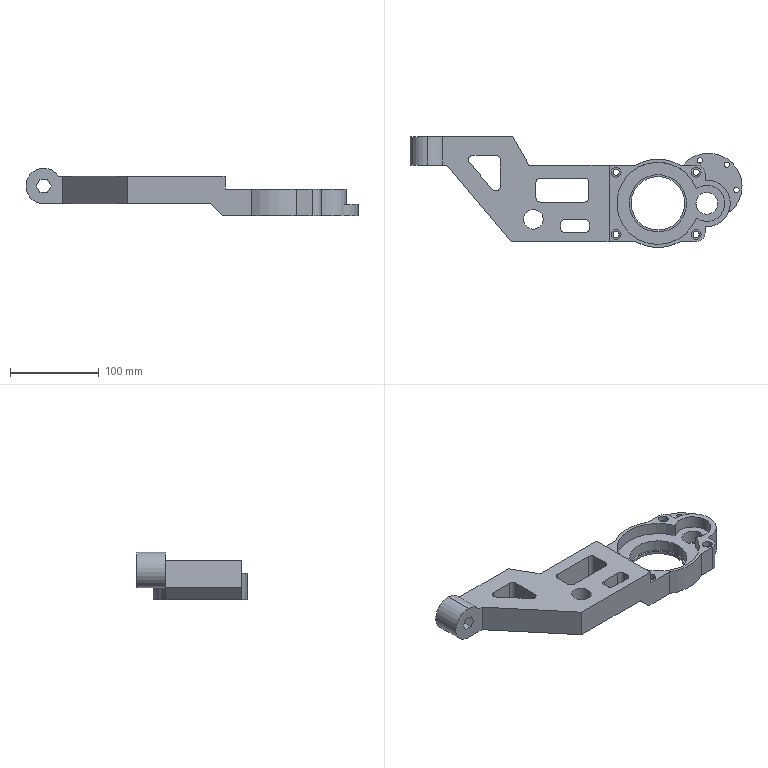Component | SolidWorks | DriveDevice-1_Bracket1-1 | 1 solid | 93 faces | volume 593022 mm3 | cylinder 53 | plane 40 | commonest cylinder face diameters 10 x11 11 x8 7 x8 6 x6 60.2 x2 40.6 x2 40 x2 52.6 x2